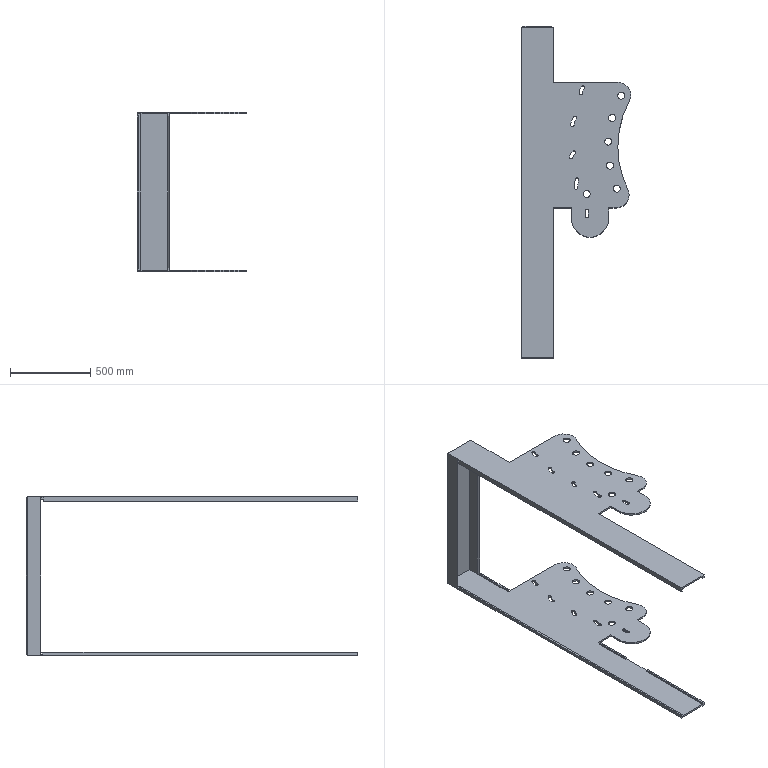Component | SolidWorks | SupportFrame-2 | 1 solid | 147 faces | volume 19548203 mm3 | cylinder 88 | plane 59 | commonest cylinder face diameters 44.189 x20 21.075 x6 22.239 x6 21.048 x6 20.03 x6 189.951 x4 233.006 x4 44.19 x4